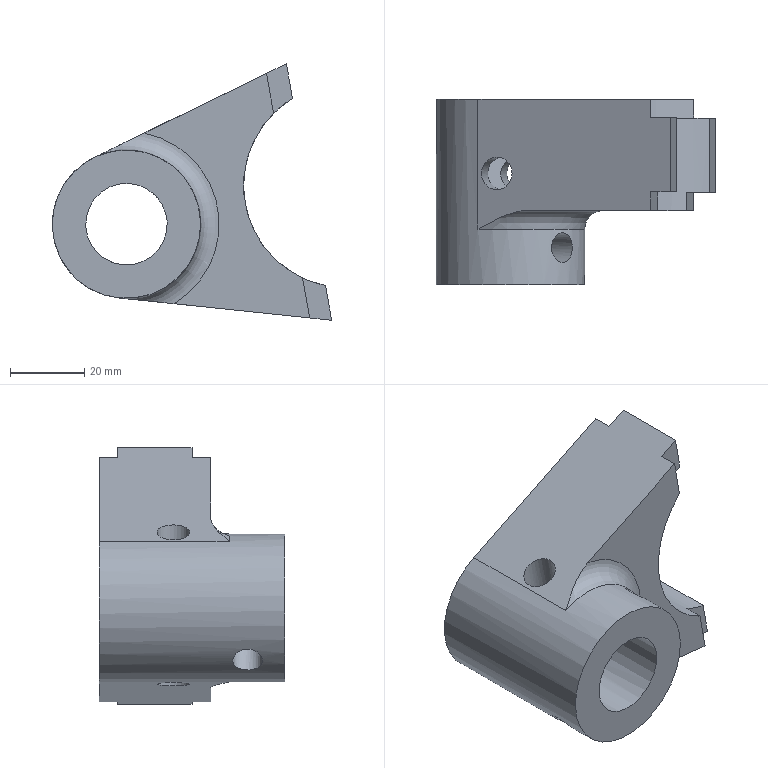Component | NX | MODEL3 | 1 solid | 23 faces | volume 83456 mm3 | plane 14 | cylinder 8 | torus 1 | commonest cylinder face diameters 8.8 x2 8 x2 73.027 x1 55 x1 40 x1 22 x1